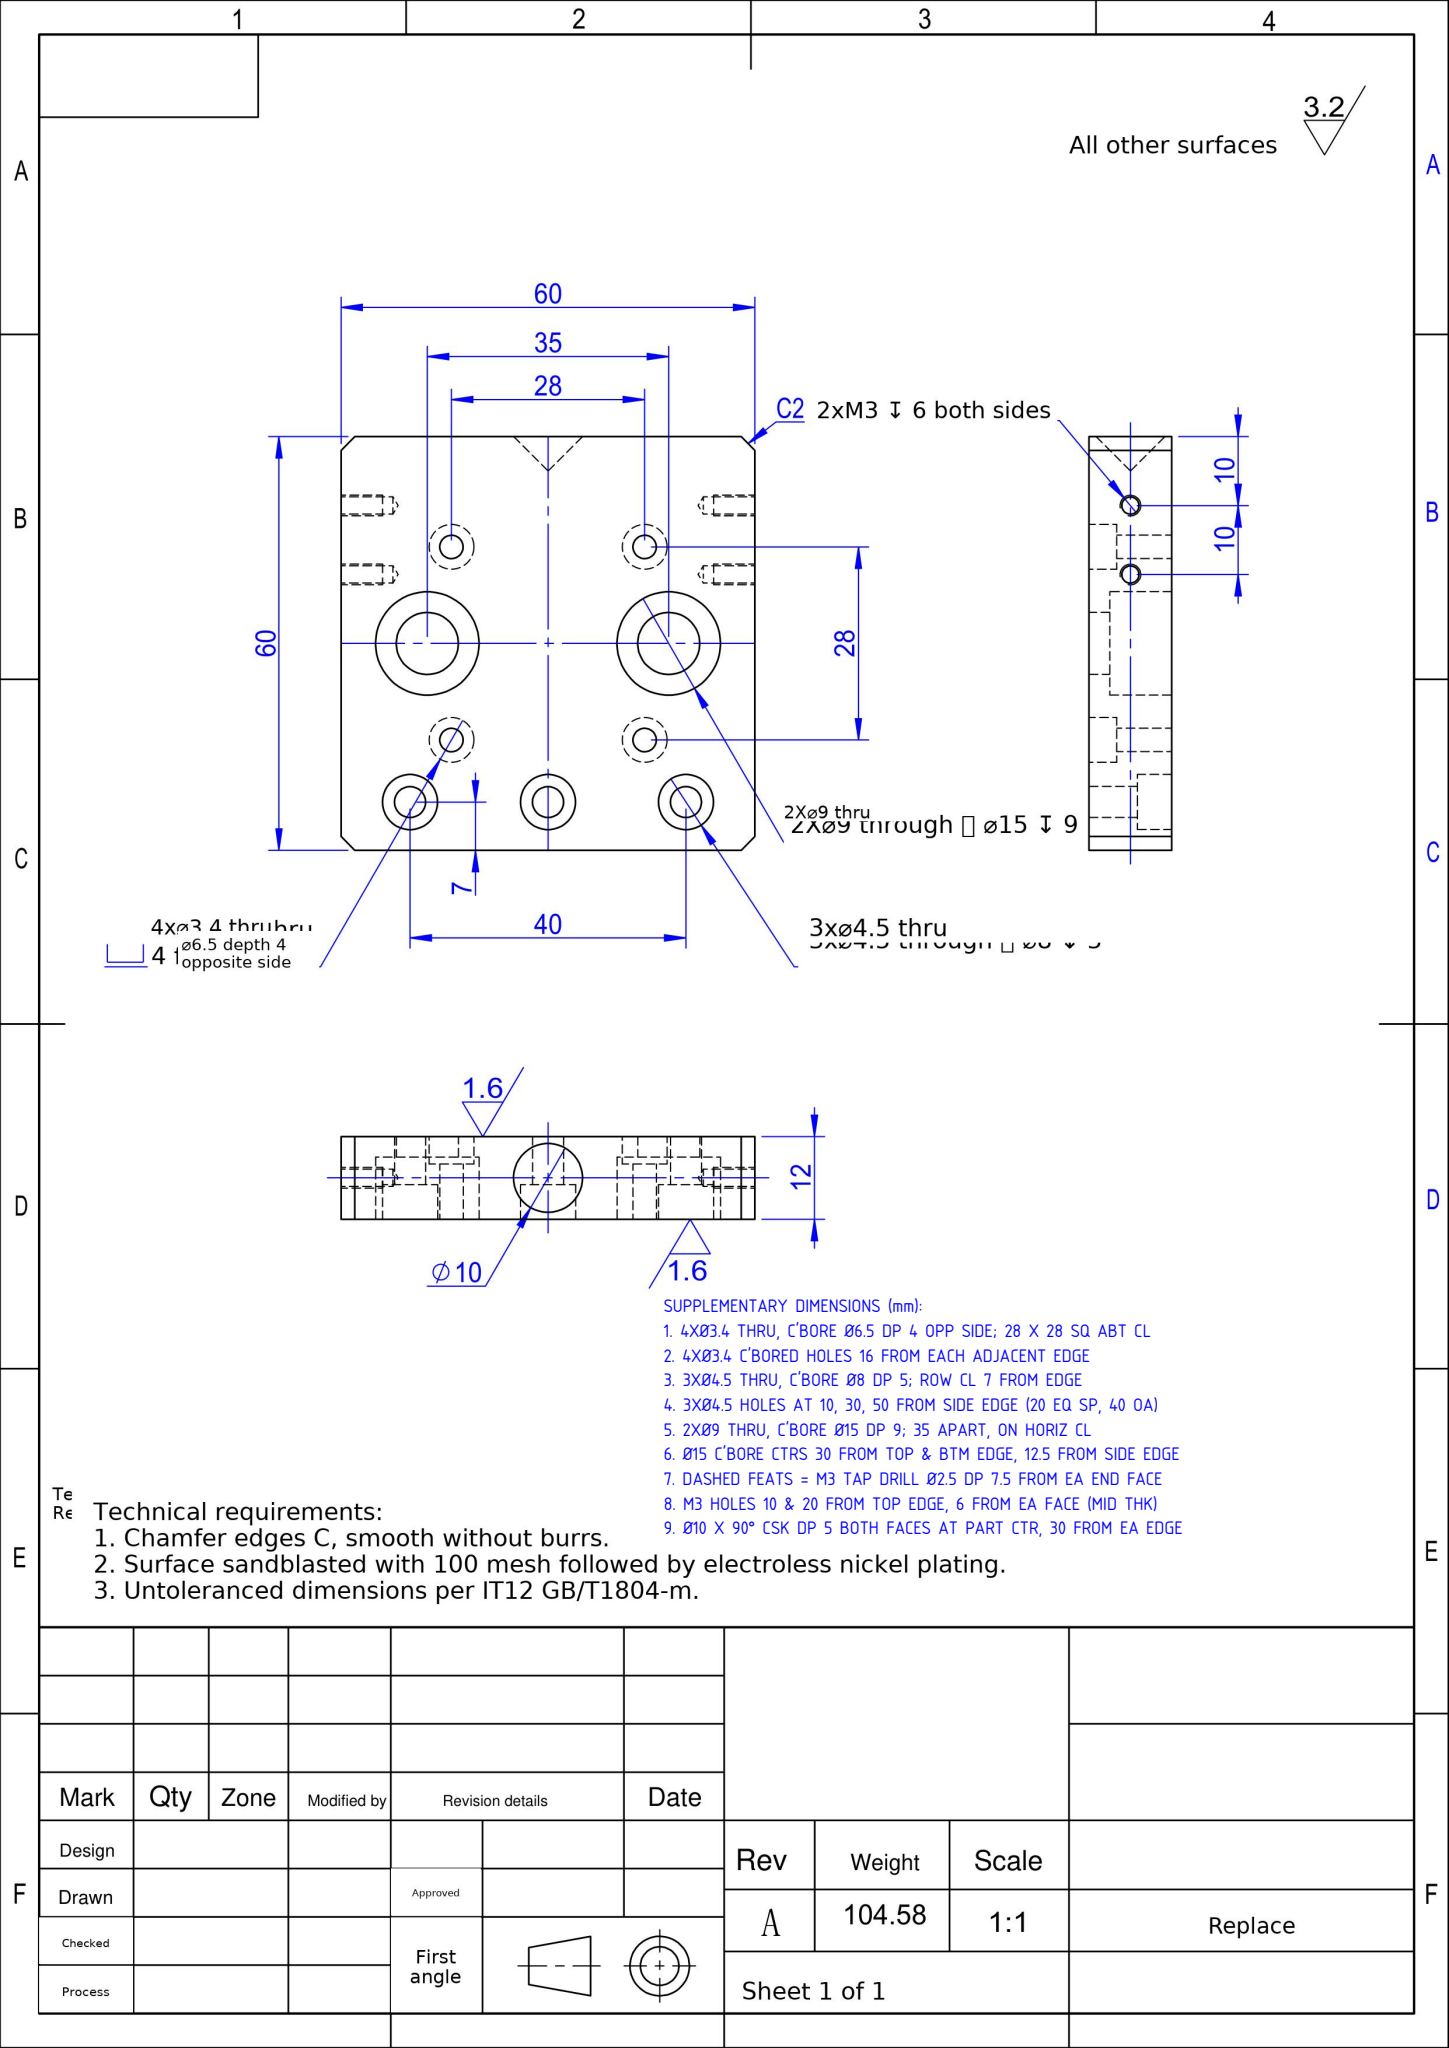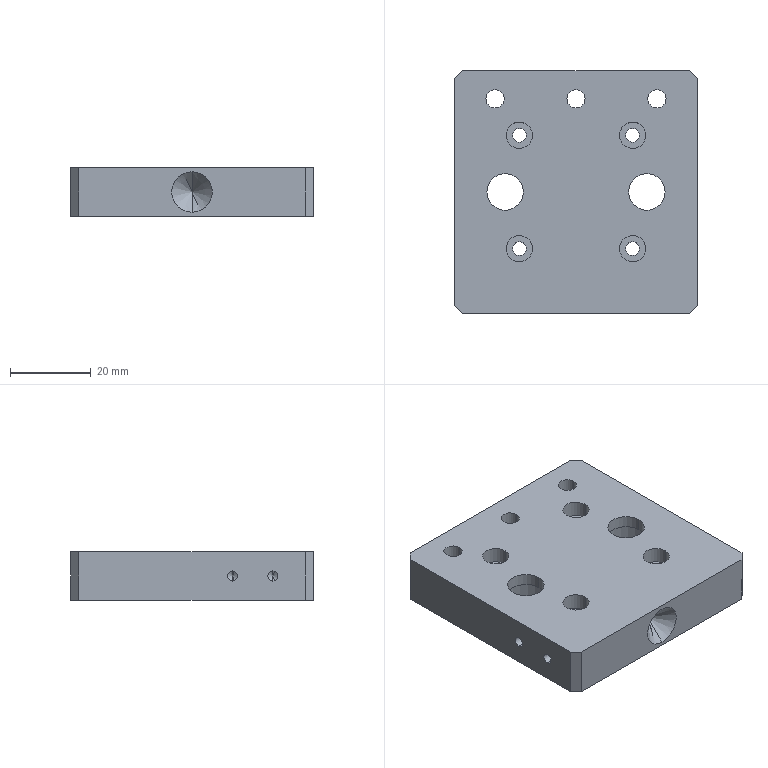Part | SolidWorks | mm | 1 solid | 73 faces | box 60 x 60 x 12 mm | volume 37349 mm3 | cylinder 44 | plane 19 | cone 10 | commonest cylinder face diameters 2.5 x8 6.5 x8 3.4 x8 8 x6 4.5 x6 15 x4 9 x4
build123d program:
from build123d import *

# Parameters (mm, degrees)
SKETCH1_W                                       = 60
SKETCH1_H                                       = 60
BOSS_EXTRUDE1_DEPTH                             = 6
M3_HEX_SOCKET_HEAD_CAP_SCREW_CBORE1_D           = 3.4
M3_HEX_SOCKET_HEAD_CAP_SCREW_CBORE1_CBORE_D     = 6.5
M3_HEX_SOCKET_HEAD_CAP_SCREW_CBORE1_CBORE_DEPTH = 4
CHAMFER1_SIZE                                   = 2
M8_HEX_SOCKET_HEAD_CAP_SCREW_CBORE1_D           = 9
M8_HEX_SOCKET_HEAD_CAP_SCREW_CBORE1_CBORE_D     = 15
M8_HEX_SOCKET_HEAD_CAP_SCREW_CBORE1_CBORE_DEPTH = 9
M4_HEX_SOCKET_HEAD_CAP_SCREW_CBORE1_D           = 4.5
M4_HEX_SOCKET_HEAD_CAP_SCREW_CBORE1_CBORE_D     = 8
M4_HEX_SOCKET_HEAD_CAP_SCREW_CBORE1_CBORE_DEPTH = 5
M3_TAPPED_HOLE1_AT_2_COUNT                      = 2
M3_TAPPED_HOLE1_AT_2_PITCH                      = 10


with BuildPart() as part:
    # Sketch1 → Boss-Extrude1 (new, symmetric)
    with BuildSketch(Plane.XY):
        Rectangle(SKETCH1_W, SKETCH1_H)
    extrude(amount=BOSS_EXTRUDE1_DEPTH, both=True)

    # M3 Hex Socket Head Cap Screw CBORE1 (through all)
    with Locations(Plane.XY.offset(6)):
        with Locations((-14, 14), (14, 14), (-14, -14), (14, -14)):
            CounterBoreHole(M3_HEX_SOCKET_HEAD_CAP_SCREW_CBORE1_D / 2, M3_HEX_SOCKET_HEAD_CAP_SCREW_CBORE1_CBORE_D / 2, M3_HEX_SOCKET_HEAD_CAP_SCREW_CBORE1_CBORE_DEPTH)

    # Chamfer1
    chamfer1_edges = [part.edges().sort_by_distance(p)[0] for p in [
        (30, -30, 0),
        (-30, -30, 0),
        (-30, 30, 0),
        (30, 30, 0),
    ]]
    chamfer(chamfer1_edges, length=CHAMFER1_SIZE)

    # M8 Hex Socket Head Cap Screw CBORE1 (through all)
    with Locations(Plane(origin=(0, 0, -6), x_dir=(-1, 0, 0), z_dir=(0, 0, -1))):
        with Locations((17.5, 0)):
            m8_hex_socket_head_cap_screw_cbore1 = CounterBoreHole(M8_HEX_SOCKET_HEAD_CAP_SCREW_CBORE1_D / 2, M8_HEX_SOCKET_HEAD_CAP_SCREW_CBORE1_CBORE_D / 2, M8_HEX_SOCKET_HEAD_CAP_SCREW_CBORE1_CBORE_DEPTH)

    # M4 Hex Socket Head Cap Screw CBORE1 (through all)
    with Locations(Plane(origin=(0, 0, -6), x_dir=(-1, 0, 0), z_dir=(0, 0, -1))):
        with Locations((20, 23), (-20, 23), (0, 23)):
            CounterBoreHole(M4_HEX_SOCKET_HEAD_CAP_SCREW_CBORE1_D / 2, M4_HEX_SOCKET_HEAD_CAP_SCREW_CBORE1_CBORE_D / 2, M4_HEX_SOCKET_HEAD_CAP_SCREW_CBORE1_CBORE_DEPTH)

    # Sketch6 → M3 Tapped Hole1 (revolve, cut)
    with BuildSketch(Plane(origin=(-30, -10, 0), x_dir=(0, 0, 1), z_dir=(0, 1, 0))):
        Polygon((0, 0), (0, 8.251), (1.25, 7.5), (1.25, 0), align=None)
    m3_tapped_hole1 = revolve(axis=Axis((-36.35, -10, 0), (1, 0, 0)), mode=Mode.SUBTRACT)

    # M3 Tapped Hole1 at 2: M3 Tapped Hole1 ×2
    with Locations(*[(0, -i * M3_TAPPED_HOLE1_AT_2_PITCH, 0) for i in range(1, M3_TAPPED_HOLE1_AT_2_COUNT)]):
        add(m3_tapped_hole1, mode=Mode.SUBTRACT)

    # Mirror1: M3 Tapped Hole1 across plane
    add(m3_tapped_hole1.mirror(Plane(origin=(0, 0, 0), x_dir=(0, 0, 1), z_dir=(1, 0, 0))), mode=Mode.SUBTRACT)

    # Mirror1 copy 1 sketch → Mirror1 copy 1 (revolve, cut)
    with BuildSketch(Plane(origin=(30, -20, 0), x_dir=(0, 0, 1), z_dir=(0, 1, 0))):
        Polygon((0, 0), (0, -8.251), (1.25, -7.5), (1.25, 0), align=None)
    revolve(axis=Axis((36.35, -20, 0), (1, 0, 0)), mode=Mode.SUBTRACT)

    # Cut-Extrude1 cone 1 section (on through the dimple's axis) → Cut-Extrude1 (revolve, cut)
    with BuildSketch(Plane(origin=(0, -30, 0), x_dir=(0, 0, -1), z_dir=(1, 0, 0))):
        Polygon((0, 0), (5, 0), (0, 5), align=None)
    revolve(axis=Axis((0, -30, 0), (0, 1, 0)), mode=Mode.SUBTRACT)

    # Mirror2: M8 Hex Socket Head Cap Screw CBORE1 across plane
    add(m8_hex_socket_head_cap_screw_cbore1.mirror(Plane(origin=(0, 0, 0), x_dir=(0, 0, 1), z_dir=(1, 0, 0))), mode=Mode.SUBTRACT)


solid = part.part